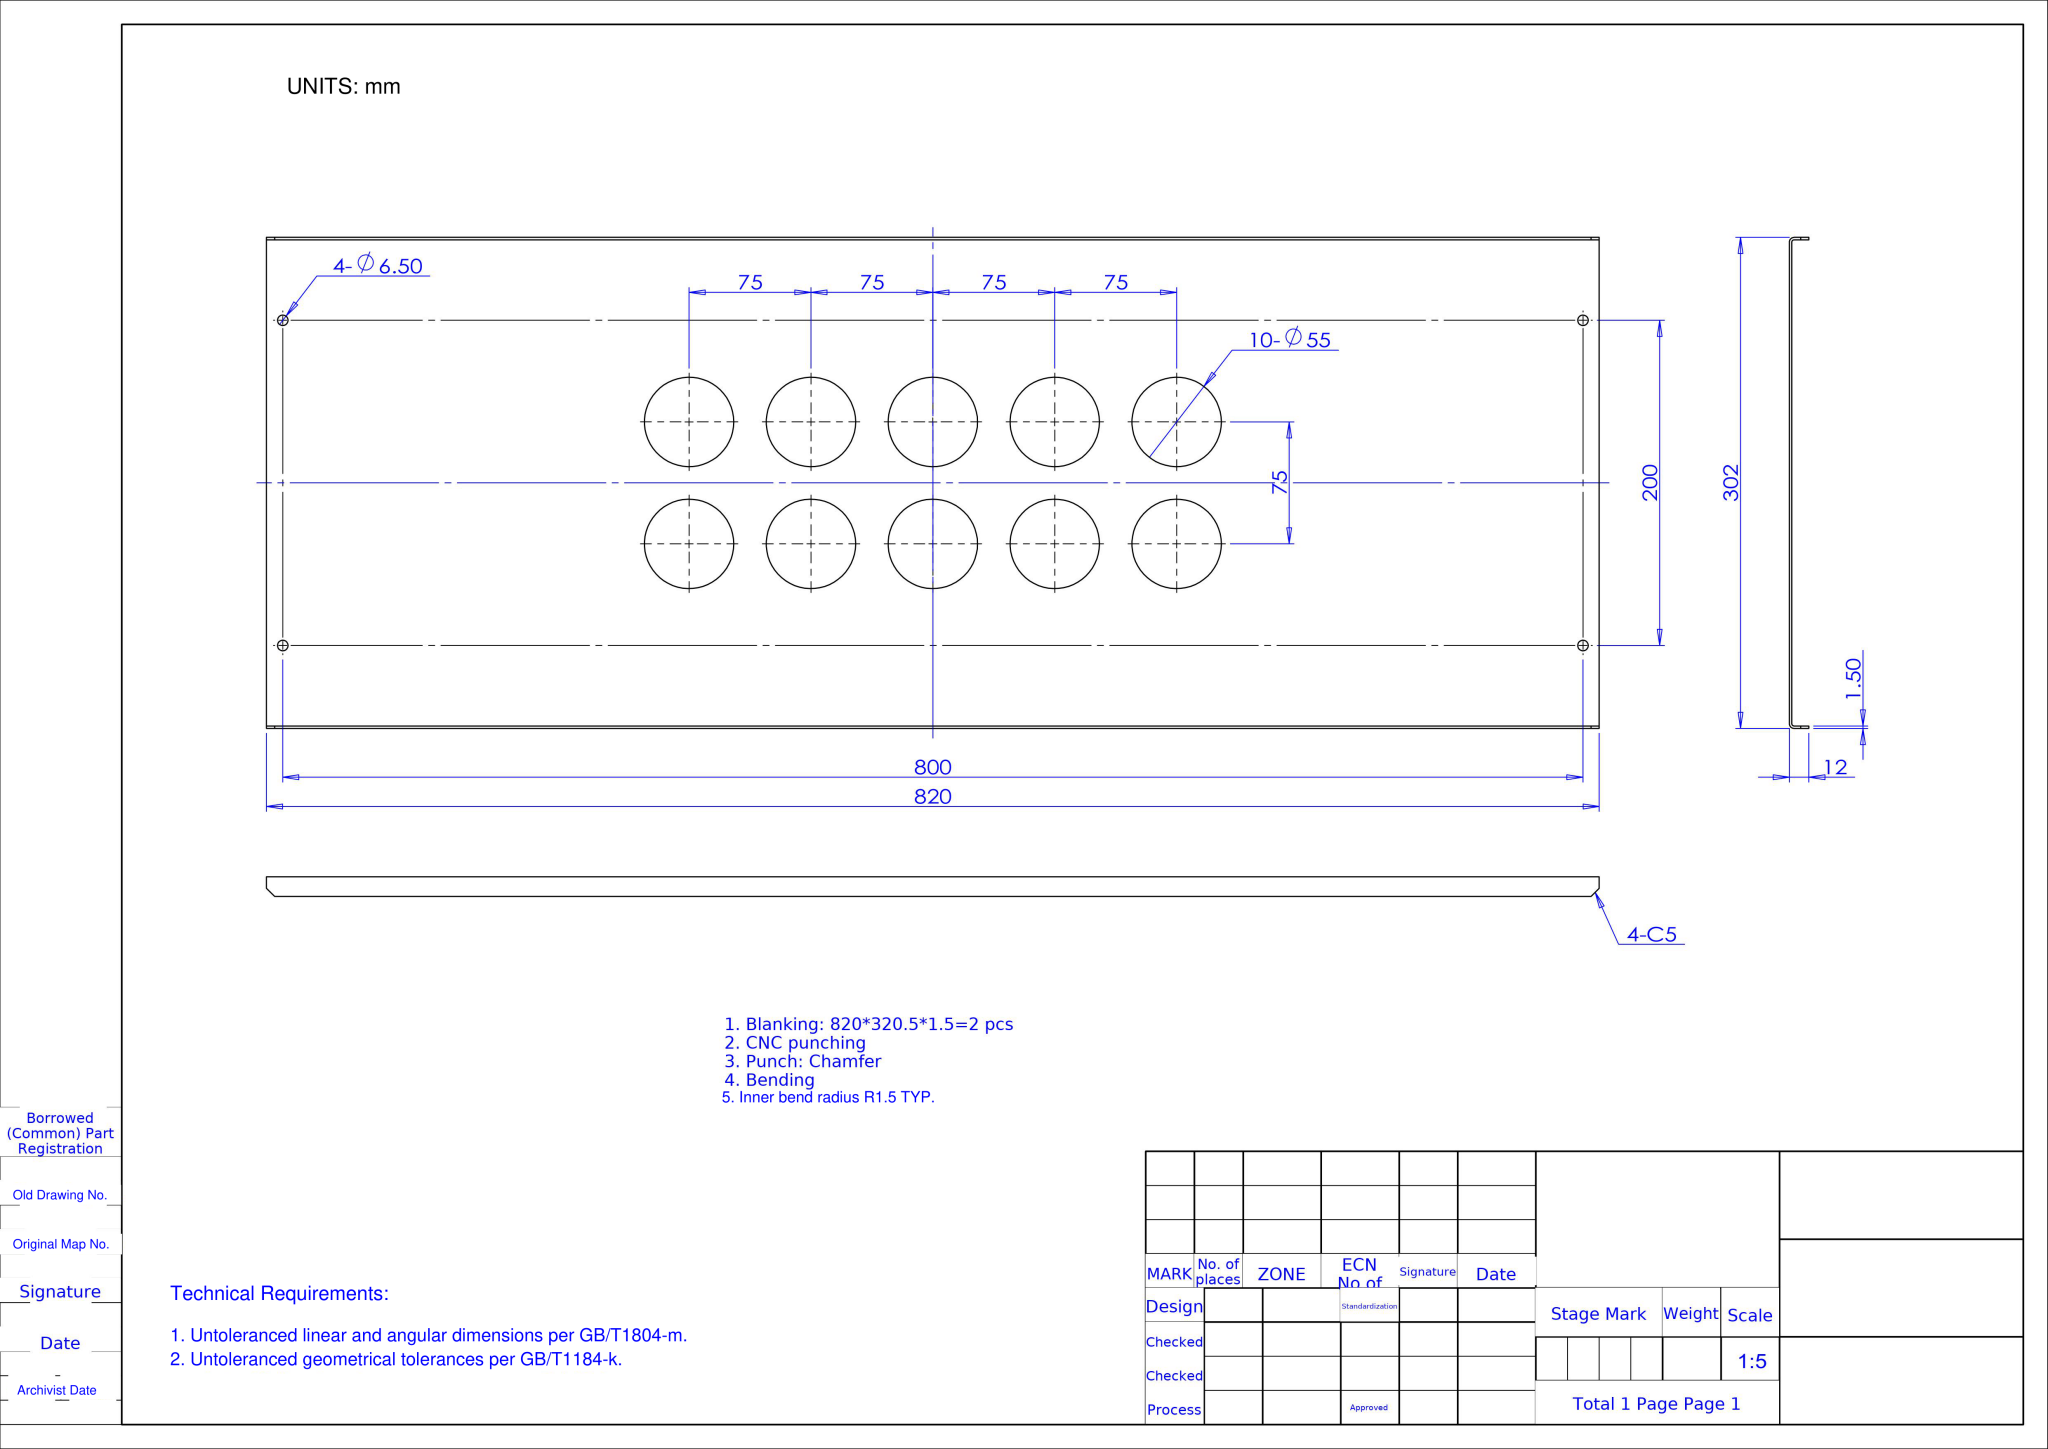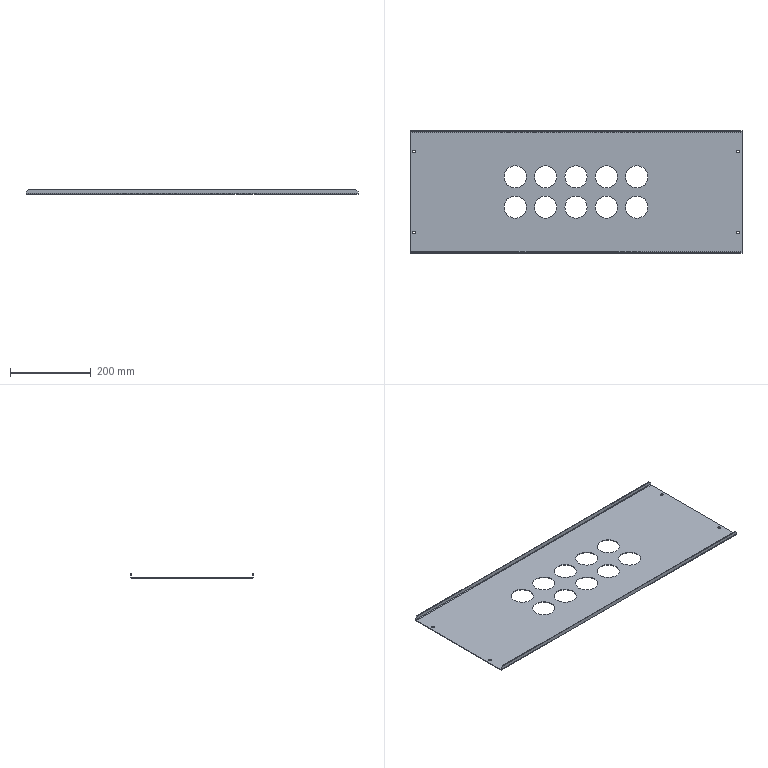Part | NX | mm | 1 solid | 54 faces | box 820 x 302 x 12 mm | volume 359003 mm3 | cylinder 32 | plane 22 | commonest cylinder face diameters 55 x20 6.5 x8 6 x2 3 x2